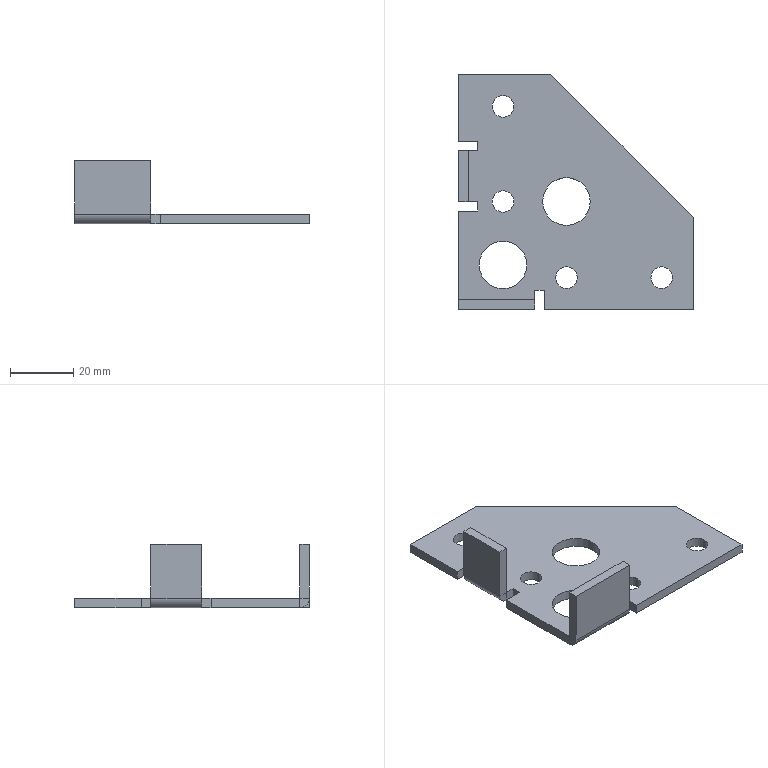Component | SolidWorks | ReinforcementPlate1-1 | 1 solid | 45 faces | volume 13695 mm3 | plane 31 | cylinder 14 | commonest cylinder face diameters 6.8 x8 15 x4 6 x2